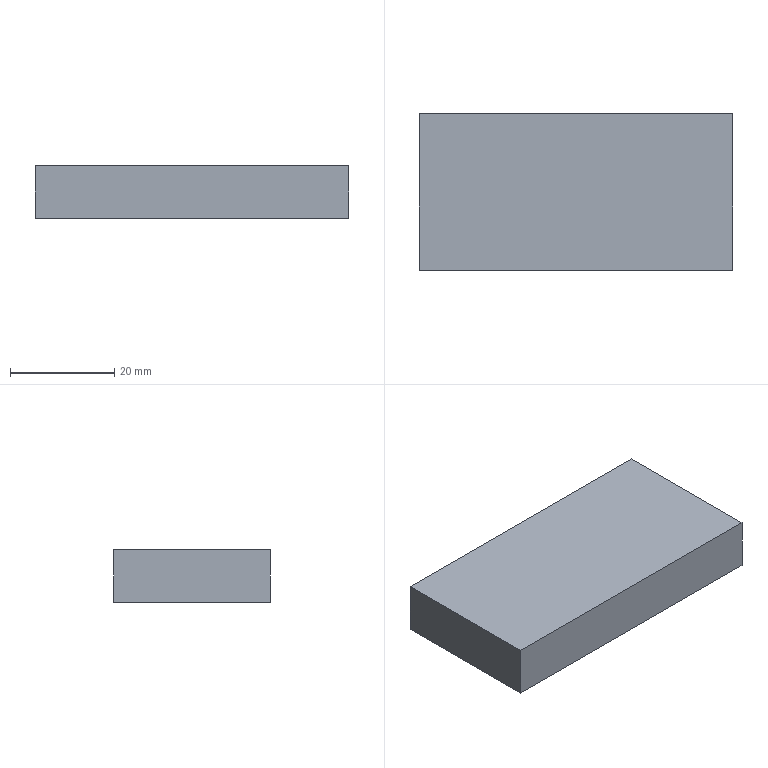Component | SolidWorks | Part48-2 | 1 solid | 6 faces | box 60 x 30 x 10 mm | volume 18000 mm3 | plane 6
build123d program:
from build123d import *

# Parameters (mm, degrees)
SKETCH1_W           = 30
SKETCH1_H           = 60
BOSS_EXTRUDE1_DEPTH = 10


with BuildPart() as part:
    # Sketch1 → Boss-Extrude1 (new body)
    with BuildSketch(Plane.XY):
        Rectangle(SKETCH1_W, SKETCH1_H)
    extrude(amount=BOSS_EXTRUDE1_DEPTH)


solid = part.part

# Placed as in the assembly
solid = solid.moved(Location((-87.007, 404, -395), (0, 0, 90)))
STEP:
#1=CARTESIAN_POINT('',(-2.244,16.496,-15.551));
#2=VERTEX_POINT('',#1);
#3=CARTESIAN_POINT('',(-4.607,16.496,-15.551));
#4=VERTEX_POINT('',#3);
#5=CARTESIAN_POINT('',(-2.244,16.496,-15.551));
#6=DIRECTION('',(-1.,0.,0.));
#7=VECTOR('',#6,39.37);
#8=LINE('',#5,#7);
#9=EDGE_CURVE('',#2,#4,#8,.T.);
#10=ORIENTED_EDGE('',*,*,#9,.T.);
#11=CARTESIAN_POINT('',(-4.607,16.496,-15.157));
#12=VERTEX_POINT('',#11);
#13=CARTESIAN_POINT('',(-4.607,16.496,-15.157));
#14=DIRECTION('',(0.,0.,-1.));
#15=VECTOR('',#14,39.37);
#16=LINE('',#13,#15);
#17=EDGE_CURVE('',#12,#4,#16,.T.);
#18=ORIENTED_EDGE('',*,*,#17,.F.);
#19=CARTESIAN_POINT('',(-2.244,16.496,-15.157));
#20=VERTEX_POINT('',#19);
#21=CARTESIAN_POINT('',(-2.244,16.496,-15.157));
#22=DIRECTION('',(-1.,0.,0.));
#23=VECTOR('',#22,39.37);
#24=LINE('',#21,#23);
#25=EDGE_CURVE('',#20,#12,#24,.T.);
#26=ORIENTED_EDGE('',*,*,#25,.F.);
#27=CARTESIAN_POINT('',(-2.244,16.496,-15.157));
#28=DIRECTION('',(0.,0.,-1.));
#29=VECTOR('',#28,39.37);
#30=LINE('',#27,#29);
#31=EDGE_CURVE('',#20,#2,#30,.T.);
#32=ORIENTED_EDGE('',*,*,#31,.T.);
#33=EDGE_LOOP('',(#10,#18,#26,#32));
#34=FACE_OUTER_BOUND('',#33,.T.);
#35=CARTESIAN_POINT('',(-2.244,16.496,-15.157));
#36=DIRECTION('',(0.,-1.,-0.));
#37=DIRECTION('',(0.,-0.,1.));
#38=AXIS2_PLACEMENT_3D('',#35,#36,#37);
#39=PLANE('',#38);
#40=ADVANCED_FACE('',(#34),#39,.F.);
#41=CARTESIAN_POINT('',(-4.607,15.315,-15.551));
#42=VERTEX_POINT('',#41);
#43=CARTESIAN_POINT('',(-4.607,15.315,-15.551));
#44=DIRECTION('',(0.,-1.,-0.));
#45=VECTOR('',#44,39.37);
#46=LINE('',#43,#45);
#47=EDGE_CURVE('',#4,#42,#46,.T.);
#48=ORIENTED_EDGE('',*,*,#47,.T.);
#49=CARTESIAN_POINT('',(-4.607,15.315,-15.157));
#50=VERTEX_POINT('',#49);
#51=CARTESIAN_POINT('',(-4.607,15.315,-15.157));
#52=DIRECTION('',(0.,0.,-1.));
#53=VECTOR('',#52,39.37);
#54=LINE('',#51,#53);
#55=EDGE_CURVE('',#50,#42,#54,.T.);
#56=ORIENTED_EDGE('',*,*,#55,.F.);
#57=CARTESIAN_POINT('',(-4.607,15.315,-15.157));
#58=DIRECTION('',(0.,-1.,-0.));
#59=VECTOR('',#58,39.37);
#60=LINE('',#57,#59);
#61=EDGE_CURVE('',#12,#50,#60,.T.);
#62=ORIENTED_EDGE('',*,*,#61,.F.);
#63=ORIENTED_EDGE('',*,*,#17,.T.);
#64=EDGE_LOOP('',(#48,#56,#62,#63));
#65=FACE_OUTER_BOUND('',#64,.T.);
#66=CARTESIAN_POINT('',(-4.607,15.315,-15.157));
#67=DIRECTION('',(1.,0.,0.));
#68=DIRECTION('',(0.,0.,-1.));
#69=AXIS2_PLACEMENT_3D('',#66,#67,#68);
#70=PLANE('',#69);
#71=ADVANCED_FACE('',(#65),#70,.F.);
#72=CARTESIAN_POINT('',(-2.244,15.315,-15.551));
#73=VERTEX_POINT('',#72);
#74=CARTESIAN_POINT('',(-2.244,15.315,-15.551));
#75=DIRECTION('',(1.,0.,0.));
#76=VECTOR('',#75,39.37);
#77=LINE('',#74,#76);
#78=EDGE_CURVE('',#42,#73,#77,.T.);
#79=ORIENTED_EDGE('',*,*,#78,.T.);
#80=CARTESIAN_POINT('',(-2.244,15.315,-15.157));
#81=VERTEX_POINT('',#80);
#82=CARTESIAN_POINT('',(-2.244,15.315,-15.157));
#83=DIRECTION('',(0.,0.,-1.));
#84=VECTOR('',#83,39.37);
#85=LINE('',#82,#84);
#86=EDGE_CURVE('',#81,#73,#85,.T.);
#87=ORIENTED_EDGE('',*,*,#86,.F.);
#88=CARTESIAN_POINT('',(-2.244,15.315,-15.157));
#89=DIRECTION('',(1.,0.,0.));
#90=VECTOR('',#89,39.37);
#91=LINE('',#88,#90);
#92=EDGE_CURVE('',#50,#81,#91,.T.);
#93=ORIENTED_EDGE('',*,*,#92,.F.);
#94=ORIENTED_EDGE('',*,*,#55,.T.);
#95=EDGE_LOOP('',(#79,#87,#93,#94));
#96=FACE_OUTER_BOUND('',#95,.T.);
#97=CARTESIAN_POINT('',(-2.244,15.315,-15.157));
#98=DIRECTION('',(0.,1.,0.));
#99=DIRECTION('',(0.,0.,-1.));
#100=AXIS2_PLACEMENT_3D('',#97,#98,#99);
#101=PLANE('',#100);
#102=ADVANCED_FACE('',(#96),#101,.F.);
#103=CARTESIAN_POINT('',(-2.244,15.315,-15.551));
#104=DIRECTION('',(0.,1.,0.));
#105=VECTOR('',#104,39.37);
#106=LINE('',#103,#105);
#107=EDGE_CURVE('',#73,#2,#106,.T.);
#108=ORIENTED_EDGE('',*,*,#107,.T.);
#109=ORIENTED_EDGE('',*,*,#31,.F.);
#110=CARTESIAN_POINT('',(-2.244,15.315,-15.157));
#111=DIRECTION('',(0.,1.,0.));
#112=VECTOR('',#111,39.37);
#113=LINE('',#110,#112);
#114=EDGE_CURVE('',#81,#20,#113,.T.);
#115=ORIENTED_EDGE('',*,*,#114,.F.);
#116=ORIENTED_EDGE('',*,*,#86,.T.);
#117=EDGE_LOOP('',(#108,#109,#115,#116));
#118=FACE_OUTER_BOUND('',#117,.T.);
#119=CARTESIAN_POINT('',(-2.244,15.315,-15.157));
#120=DIRECTION('',(-1.,0.,0.));
#121=DIRECTION('',(0.,-0.,1.));
#122=AXIS2_PLACEMENT_3D('',#119,#120,#121);
#123=PLANE('',#122);
#124=ADVANCED_FACE('',(#118),#123,.F.);
#125=ORIENTED_EDGE('',*,*,#25,.T.);
#126=ORIENTED_EDGE('',*,*,#61,.T.);
#127=ORIENTED_EDGE('',*,*,#92,.T.);
#128=ORIENTED_EDGE('',*,*,#114,.T.);
#129=EDGE_LOOP('',(#125,#126,#127,#128));
#130=FACE_OUTER_BOUND('',#129,.T.);
#131=CARTESIAN_POINT('',(-3.425,15.906,-15.157));
#132=DIRECTION('',(0.,0.,-1.));
#133=DIRECTION('',(0.,-1.,-0.));
#134=AXIS2_PLACEMENT_3D('',#131,#132,#133);
#135=PLANE('',#134);
#136=ADVANCED_FACE('',(#130),#135,.F.);
#137=ORIENTED_EDGE('',*,*,#9,.F.);
#138=ORIENTED_EDGE('',*,*,#107,.F.);
#139=ORIENTED_EDGE('',*,*,#78,.F.);
#140=ORIENTED_EDGE('',*,*,#47,.F.);
#141=EDGE_LOOP('',(#137,#138,#139,#140));
#142=FACE_OUTER_BOUND('',#141,.T.);
#143=CARTESIAN_POINT('',(-3.425,15.906,-15.551));
#144=DIRECTION('',(0.,0.,-1.));
#145=DIRECTION('',(0.,-1.,-0.));
#146=AXIS2_PLACEMENT_3D('',#143,#144,#145);
#147=PLANE('',#146);
#148=ADVANCED_FACE('',(#142),#147,.T.);
#149=CLOSED_SHELL('',(#40,#71,#102,#124,#136,#148));
#150=MANIFOLD_SOLID_BREP('',#149);
#151=CARTESIAN_POINT('',(0.,0.,0.));
#152=DIRECTION('',(0.,0.,1.));
#153=DIRECTION('',(1.,0.,0.));
#154=AXIS2_PLACEMENT_3D('',#151,#152,#153);
#155=(LENGTH_UNIT()NAMED_UNIT(*)SI_UNIT($,.METRE.));
#156=LENGTH_MEASURE_WITH_UNIT(LENGTH_MEASURE(0.0254),#155);
#157=DIMENSIONAL_EXPONENTS(1.,0.,0.,0.,0.,0.,0.);
#158=(CONVERSION_BASED_UNIT('',#156)LENGTH_UNIT()NAMED_UNIT(#157));
#159=UNCERTAINTY_MEASURE_WITH_UNIT(LENGTH_MEASURE(0.00001),#158,'','');
#160=(NAMED_UNIT(*)PLANE_ANGLE_UNIT()SI_UNIT($,.RADIAN.));
#161=(NAMED_UNIT(*)SI_UNIT($,.STERADIAN.)SOLID_ANGLE_UNIT());
#162=(GEOMETRIC_REPRESENTATION_CONTEXT(3)GLOBAL_UNCERTAINTY_ASSIGNED_CONTEXT((#159))GLOBAL_UNIT_ASSIGNED_CONTEXT((#158,#160,#161))REPRESENTATION_CONTEXT('',''));
#163=ADVANCED_BREP_SHAPE_REPRESENTATION('',(#150,#154),#162);
#164=COLOUR_RGB('',0.7922,0.8196,0.9333);
#165=FILL_AREA_STYLE_COLOUR('',#164);
#166=FILL_AREA_STYLE('',(#165));
#167=SURFACE_STYLE_FILL_AREA(#166);
#168=SURFACE_SIDE_STYLE('',(#167));
#169=SURFACE_STYLE_USAGE(.BOTH.,#168);
#170=PRESENTATION_STYLE_ASSIGNMENT((#169));
#171=STYLED_ITEM('',(#170),#150);
#172=PRESENTATION_LAYER_ASSIGNMENT('','',(#171));
#173=(LENGTH_UNIT()NAMED_UNIT(*)SI_UNIT($,.METRE.));
#174=LENGTH_MEASURE_WITH_UNIT(LENGTH_MEASURE(0.0254),#173);
#175=DIMENSIONAL_EXPONENTS(1.,0.,0.,0.,0.,0.,0.);
#176=(CONVERSION_BASED_UNIT('',#174)LENGTH_UNIT()NAMED_UNIT(#175));
#177=UNCERTAINTY_MEASURE_WITH_UNIT(LENGTH_MEASURE(0.00001),#176,'','');
#178=(NAMED_UNIT(*)PLANE_ANGLE_UNIT()SI_UNIT($,.RADIAN.));
#179=(NAMED_UNIT(*)SI_UNIT($,.STERADIAN.)SOLID_ANGLE_UNIT());
#180=(GEOMETRIC_REPRESENTATION_CONTEXT(3)GLOBAL_UNCERTAINTY_ASSIGNED_CONTEXT((#177))GLOBAL_UNIT_ASSIGNED_CONTEXT((#176,#178,#179))REPRESENTATION_CONTEXT('',''));
#181=MECHANICAL_DESIGN_GEOMETRIC_PRESENTATION_REPRESENTATION('',(#171),#180);